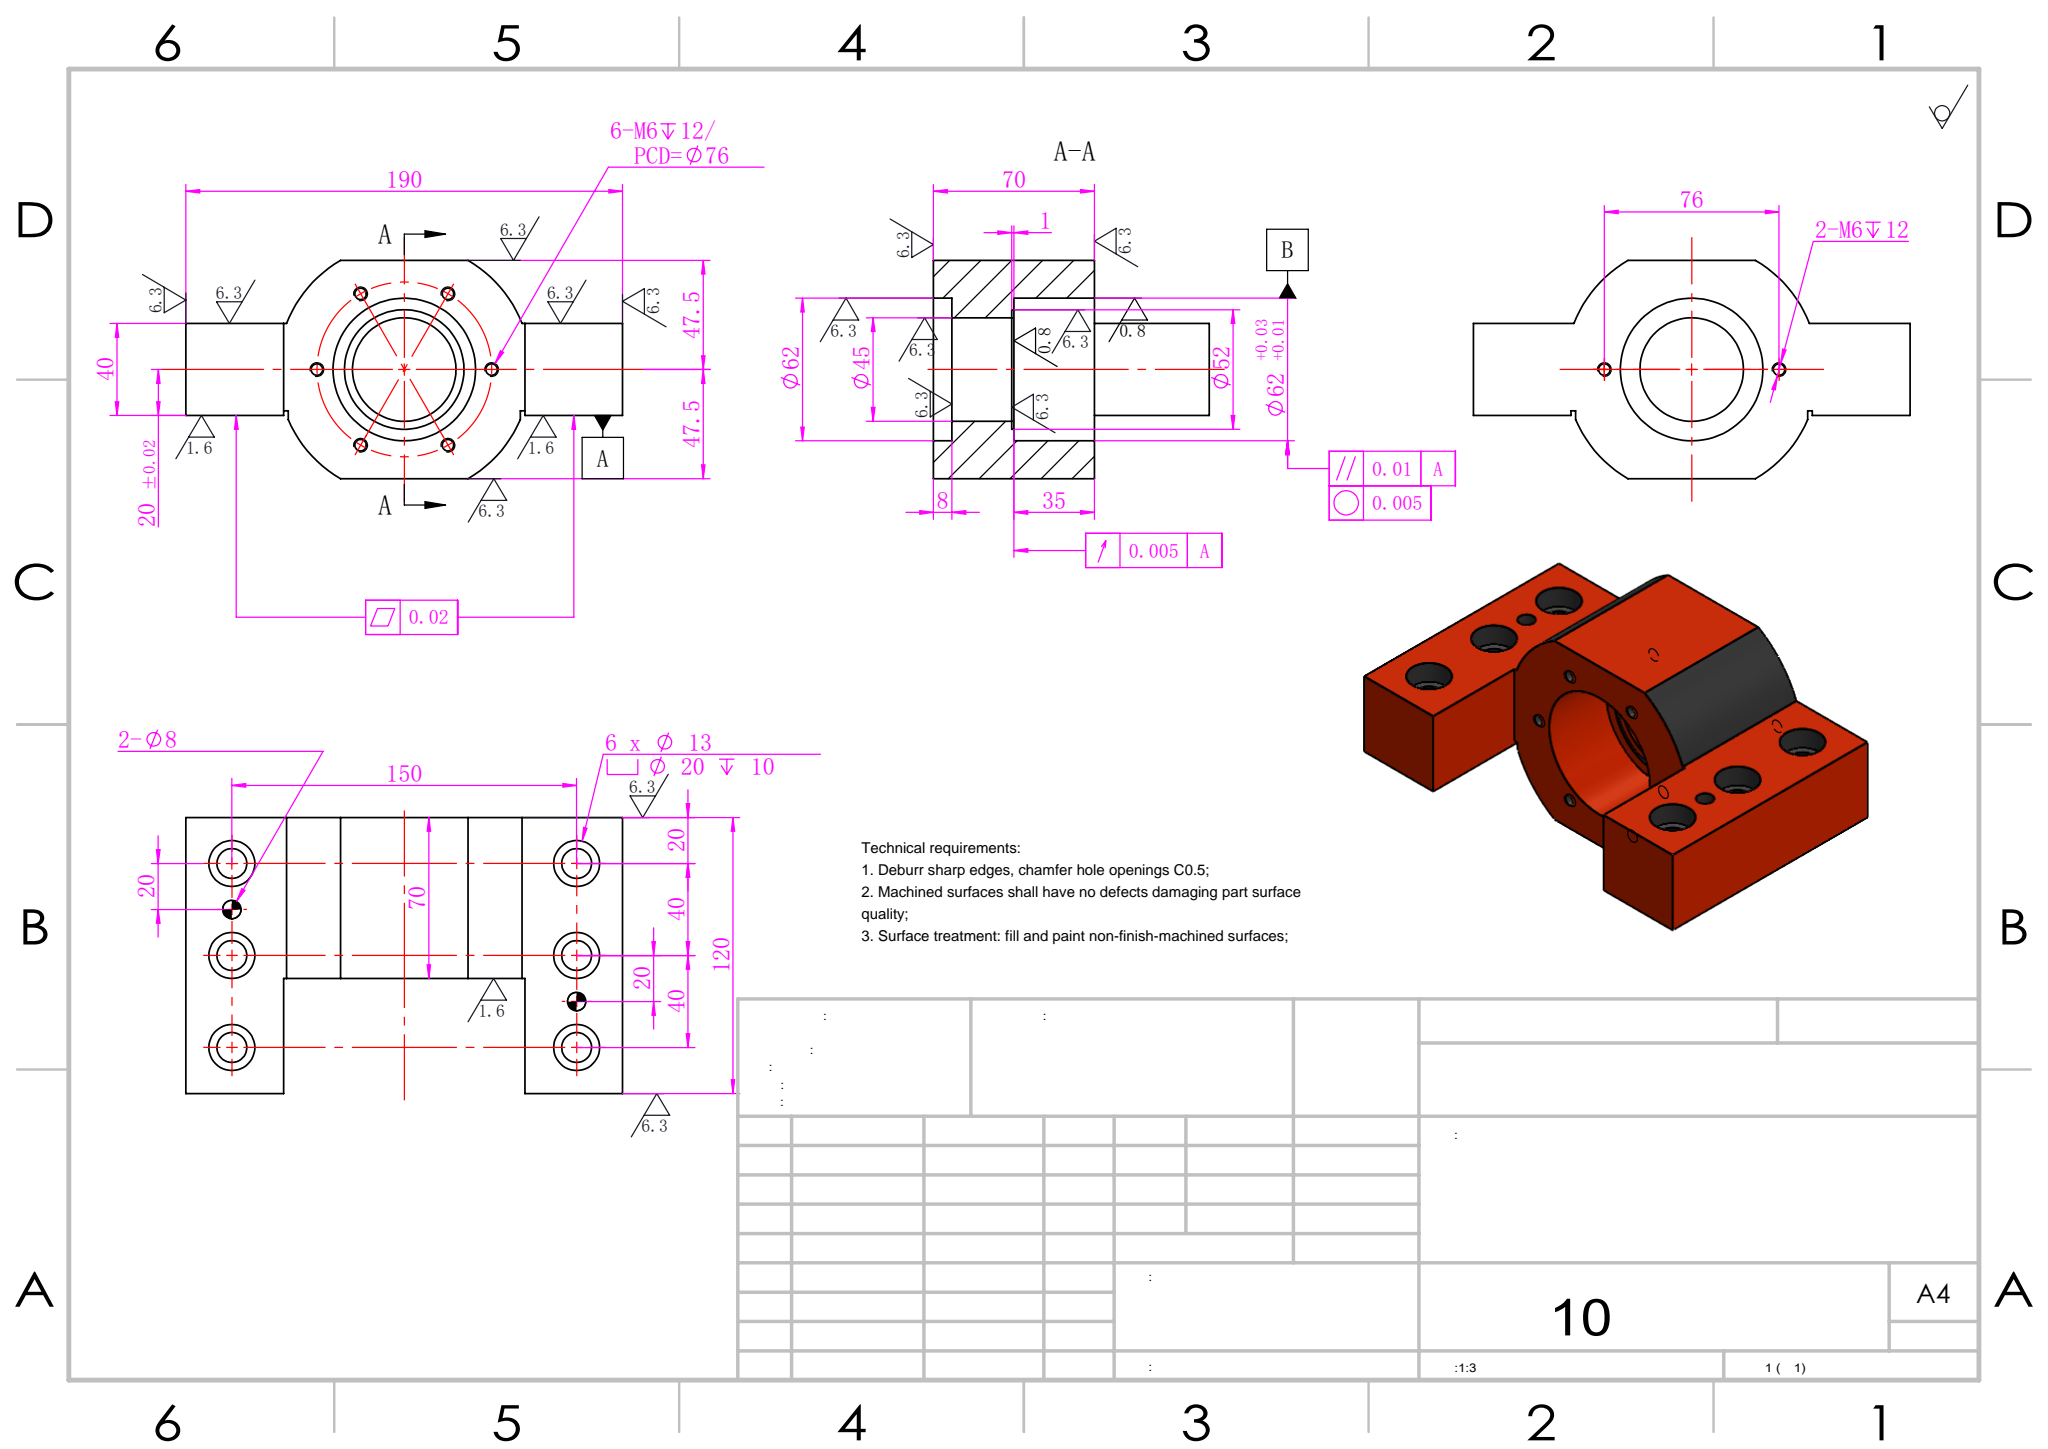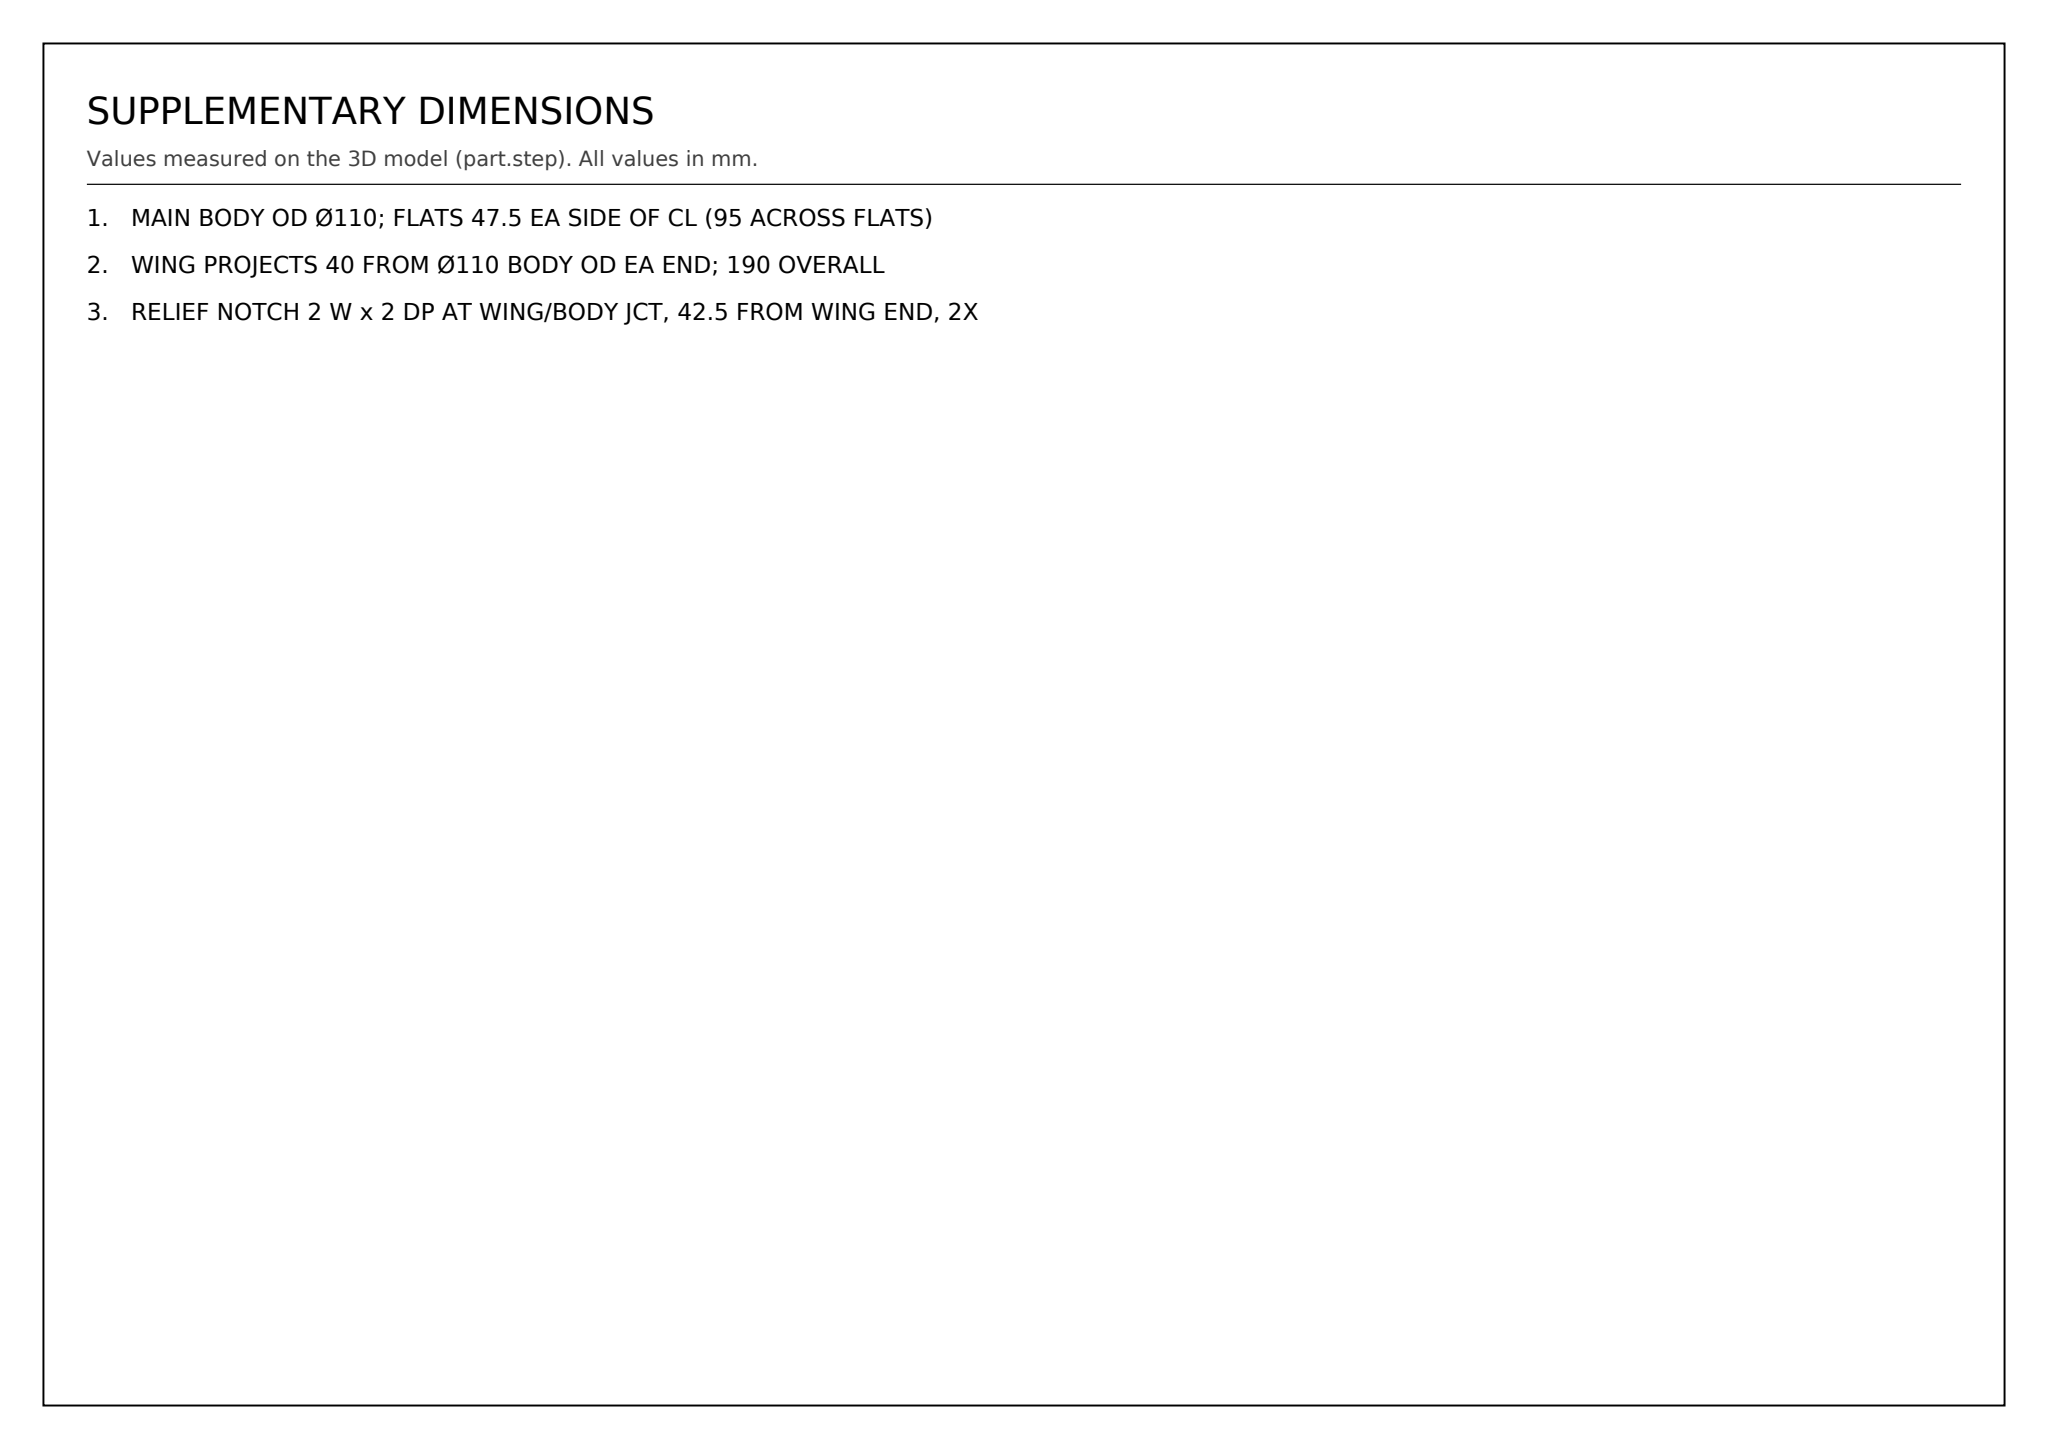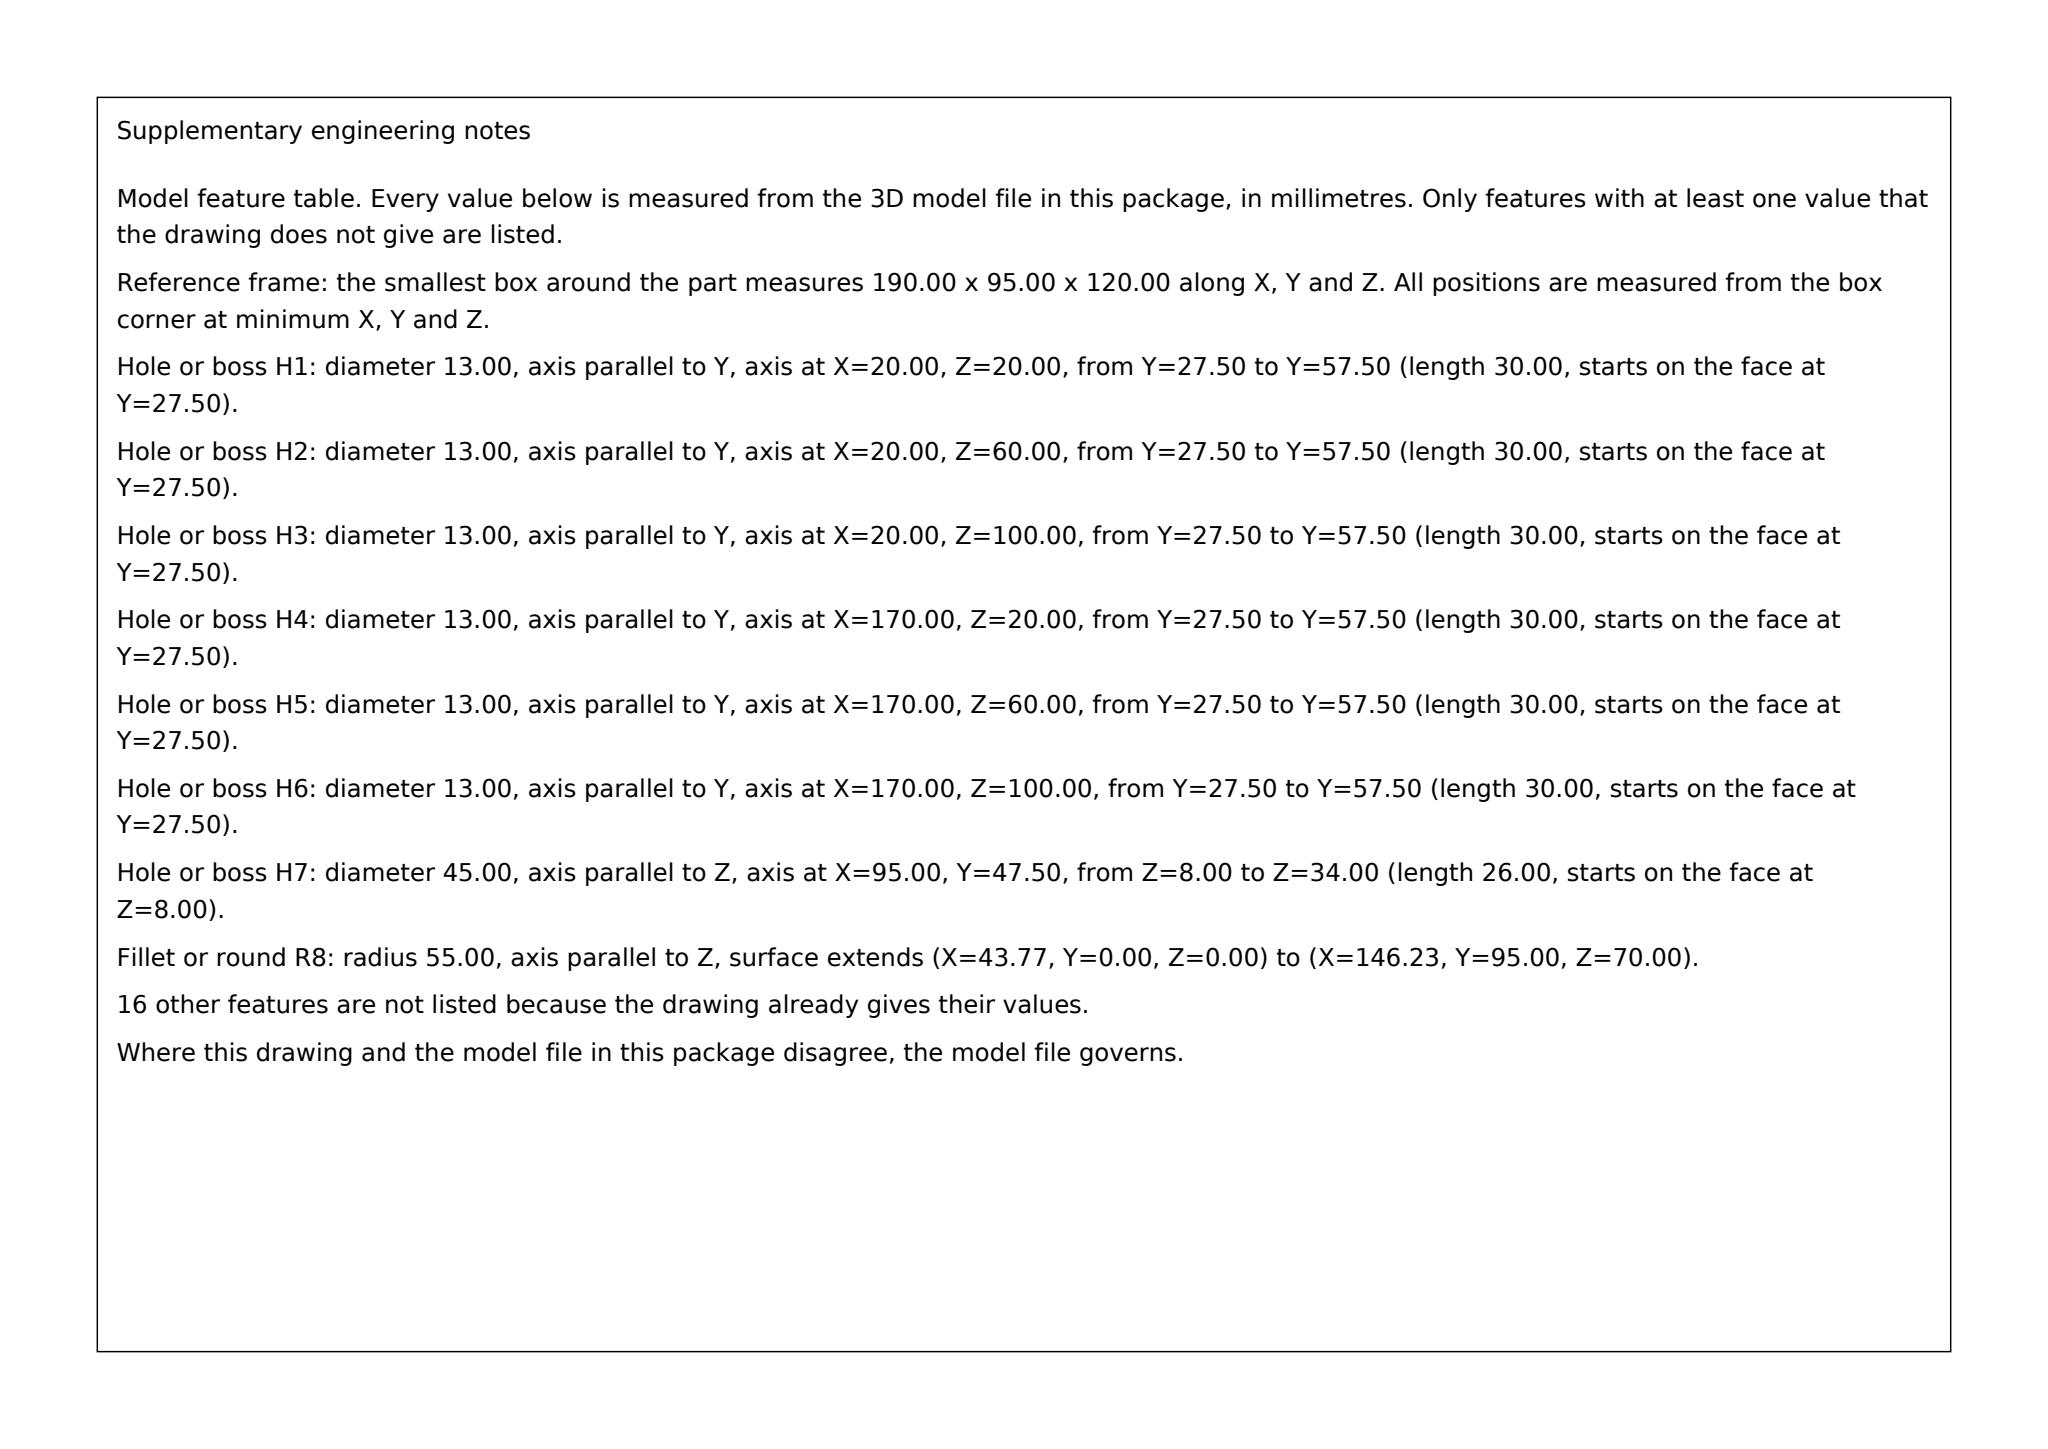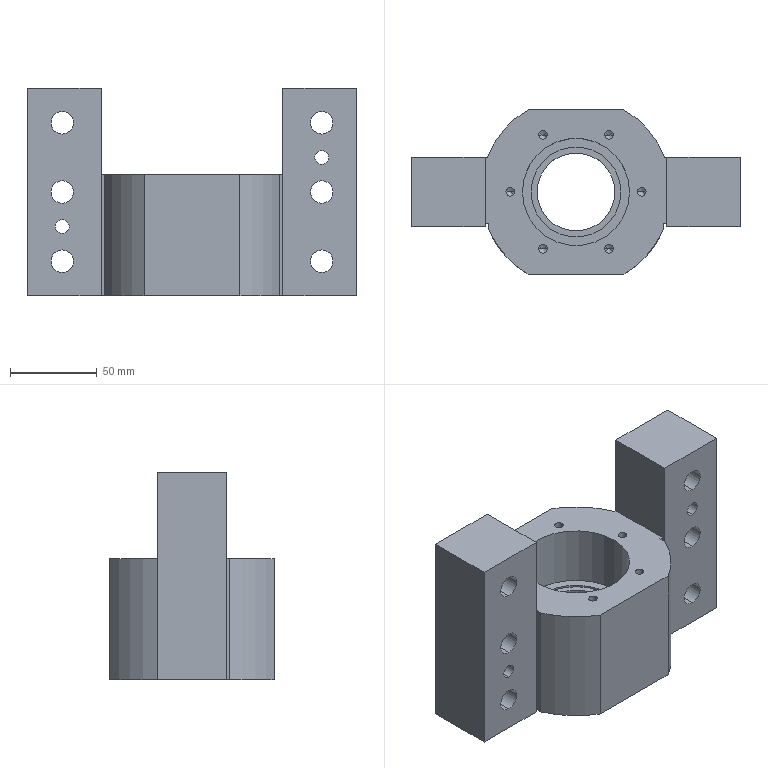Part | SolidWorks | mm | 1 solid | 99 faces | box 190 x 95 x 120 mm | volume 803165 mm3 | cylinder 56 | plane 27 | cone 16 | commonest cylinder face diameters 5 x16 20 x12 13 x12 8 x4 62 x4 110 x4 52 x2 45 x2
Drawing notes:
MAIN BODY OD Ø110; FLATS 47.5 EA SIDE OF CL (95 ACROSS FLATS) | from the solid: cylinder dia 110, axis z at (95,47.5), len 70; y-planes 0 and 95 give 47.5 ea side of CL
WING PROJECTS 40 FROM Ø110 BODY OD EA END; 190 OVERALL | from the solid: bbox x=190, body Ø110 centered x=95 -> body spans 40..150, wing 40 ea end
RELIEF NOTCH 2 W x 2 DP AT WING/BODY JCT, 42.5 FROM WING END, 2X | from the solid: x-planes 42.5/44.5 and 145.5/147.5; wing face y=27.5, notch floor y=29.5
build123d program:
from build123d import *

# Parameters (mm, degrees)
SKETCH1_R                                            = 22.5
BOSS_EXTRUDE1_DEPTH                                  = 120
SKETCH3_W                                            = 105
SKETCH3_H                                            = 150
CUT_EXTRUDE1_DEPTH                                   = 50
SKETCH4_R                                            = 31
CUT_EXTRUDE2_DEPTH                                   = 35
CUT_EXTRUDE7_START                                   = -8
SKETCH18_R                                           = 31
CUT_EXTRUDE7_DEPTH                                   = 8
SKETCH19_R                                           = 26
CUT_EXTRUDE8_DEPTH                                   = 1
CYLINDRICAL_COUNTERSUNK_HOLE_1_FOR_M12_H_D           = 13
CYLINDRICAL_COUNTERSUNK_HOLE_1_FOR_M12_H_CBORE_D     = 20
CYLINDRICAL_COUNTERSUNK_HOLE_1_FOR_M12_H_CBORE_DEPTH = 10
CIRPATTERN1_COUNT                                    = 6
SIZE_MM_DOWEL_PIN_HOLE_1_D                           = 8
SKETCH17_W                                           = 2
SKETCH17_H                                           = 20
CUT_EXTRUDE6_DEPTH                                   = 161.254
M6_TAPPED_HOLE2_D                                    = 5
M6_TAPPED_HOLE2_DEPTH                                = 18
M6_TAPPED_HOLE2_TIP                                  = 1.502


with BuildPart() as part:
    # Sketch1 → Boss-Extrude1 (new body)
    with BuildSketch(Plane.XY):
        with BuildLine():
            Line((-95, 20), (-51.235, 20))
            ThreePointArc((-51.235, 20), (-41.806, 35.738), (-27.726, 47.5))
            Line((-27.726, 47.5), (27.726, 47.5))
            ThreePointArc((27.726, 47.5), (41.806, 35.738), (51.235, 20))
            Line((51.235, 20), (95, 20))
            Line((95, 20), (95, -20))
            Line((95, -20), (51.235, -20))
            ThreePointArc((51.235, -20), (41.806, -35.738), (27.726, -47.5))
            Line((27.726, -47.5), (-27.726, -47.5))
            ThreePointArc((-27.726, -47.5), (-41.806, -35.738), (-51.235, -20))
            Line((-51.235, -20), (-95, -20))
            Line((-95, -20), (-95, 20))
        make_face()
        Circle(SKETCH1_R, mode=Mode.SUBTRACT)
    extrude(amount=BOSS_EXTRUDE1_DEPTH)

    # Sketch3 → Cut-Extrude1 (cut)
    with BuildSketch(Plane.XY.offset(120)):
        Rectangle(SKETCH3_W, SKETCH3_H)
    extrude(amount=-CUT_EXTRUDE1_DEPTH, mode=Mode.SUBTRACT)

    # Sketch4 → Cut-Extrude2 (cut)
    with BuildSketch(Plane.XY.offset(70)):
        Circle(SKETCH4_R)
    extrude(amount=-CUT_EXTRUDE2_DEPTH, mode=Mode.SUBTRACT)

    # Sketch18 → Cut-Extrude7 (cut)
    with BuildSketch(Plane(origin=(0, 0, 0), x_dir=(-1, 0, 0), z_dir=(0, 0, -1)).offset(CUT_EXTRUDE7_START)):
        with Locations(Location((0, 0, 0), (0, 0, 180))):
            Circle(SKETCH18_R)
    extrude(amount=CUT_EXTRUDE7_DEPTH, mode=Mode.SUBTRACT)

    # Sketch19 → Cut-Extrude8 (cut)
    with BuildSketch(Plane.XY.offset(35)):
        Circle(SKETCH19_R)
    extrude(amount=-CUT_EXTRUDE8_DEPTH, mode=Mode.SUBTRACT)

    # Cylindrical Countersunk Hole 1 for M12 H (through all)
    with Locations(Plane(origin=(-75, 20, 100), x_dir=(1, 0, 0), z_dir=(0, 1, 0))):
        with Locations((0, 0), (0, 40), (0, 80), (150, 0), (150, 40), (150, 80)):
            CounterBoreHole(CYLINDRICAL_COUNTERSUNK_HOLE_1_FOR_M12_H_D / 2, CYLINDRICAL_COUNTERSUNK_HOLE_1_FOR_M12_H_CBORE_D / 2, CYLINDRICAL_COUNTERSUNK_HOLE_1_FOR_M12_H_CBORE_DEPTH)

    # Sketch9 → M6 Tapped Hole1 (revolve, cut)
    with BuildSketch(Plane(origin=(38, 0, 70), x_dir=(0, -1, 0), z_dir=(1, 0, 0))):
        Polygon((0, 0), (0, 19.502), (2.5, 18), (2.5, 0), align=None)
    m6_tapped_hole1 = revolve(axis=Axis((38, 0, 76.35), (0, 0, -1)), mode=Mode.SUBTRACT)

    # CirPattern1: M6 Tapped Hole1 ×6 about axis
    cirpattern1_axis = Axis((0, 0, 0), (0, 0, 1))
    for i in range(1, CIRPATTERN1_COUNT):
        add(m6_tapped_hole1.rotate(cirpattern1_axis, i * 360 / CIRPATTERN1_COUNT), mode=Mode.SUBTRACT)

    # Size mm Dowel Pin Hole 1 (through all)
    with Locations(Plane(origin=(-75, 20, 40), x_dir=(1, 0, 0), z_dir=(0, 1, 0))):
        with Locations((0, 0), (150, -40)):
            Hole(SIZE_MM_DOWEL_PIN_HOLE_1_D / 2)

    # Sketch17 → Cut-Extrude6 (cut, through all)
    with BuildSketch(Plane.XY.offset(120)):
        with Locations((-51.5, -28)):
            Rectangle(SKETCH17_W, SKETCH17_H)
        with Locations((51.5, -28)):
            Rectangle(SKETCH17_W, SKETCH17_H)
    extrude(amount=-CUT_EXTRUDE6_DEPTH, mode=Mode.SUBTRACT)

    # M6 Tapped Hole2
    with Locations(Plane(origin=(38, 0, 0), x_dir=(-1, 0, 0), z_dir=(0, 0, -1))):
        with Locations((0, 0), (76, 0)):
            Hole(M6_TAPPED_HOLE2_D / 2, depth=M6_TAPPED_HOLE2_DEPTH)
            with Locations((0, 0, -(M6_TAPPED_HOLE2_DEPTH + M6_TAPPED_HOLE2_TIP / 2))):  # 118° drill point
                Cone(0, M6_TAPPED_HOLE2_D / 2, M6_TAPPED_HOLE2_TIP, mode=Mode.SUBTRACT)


solid = part.part